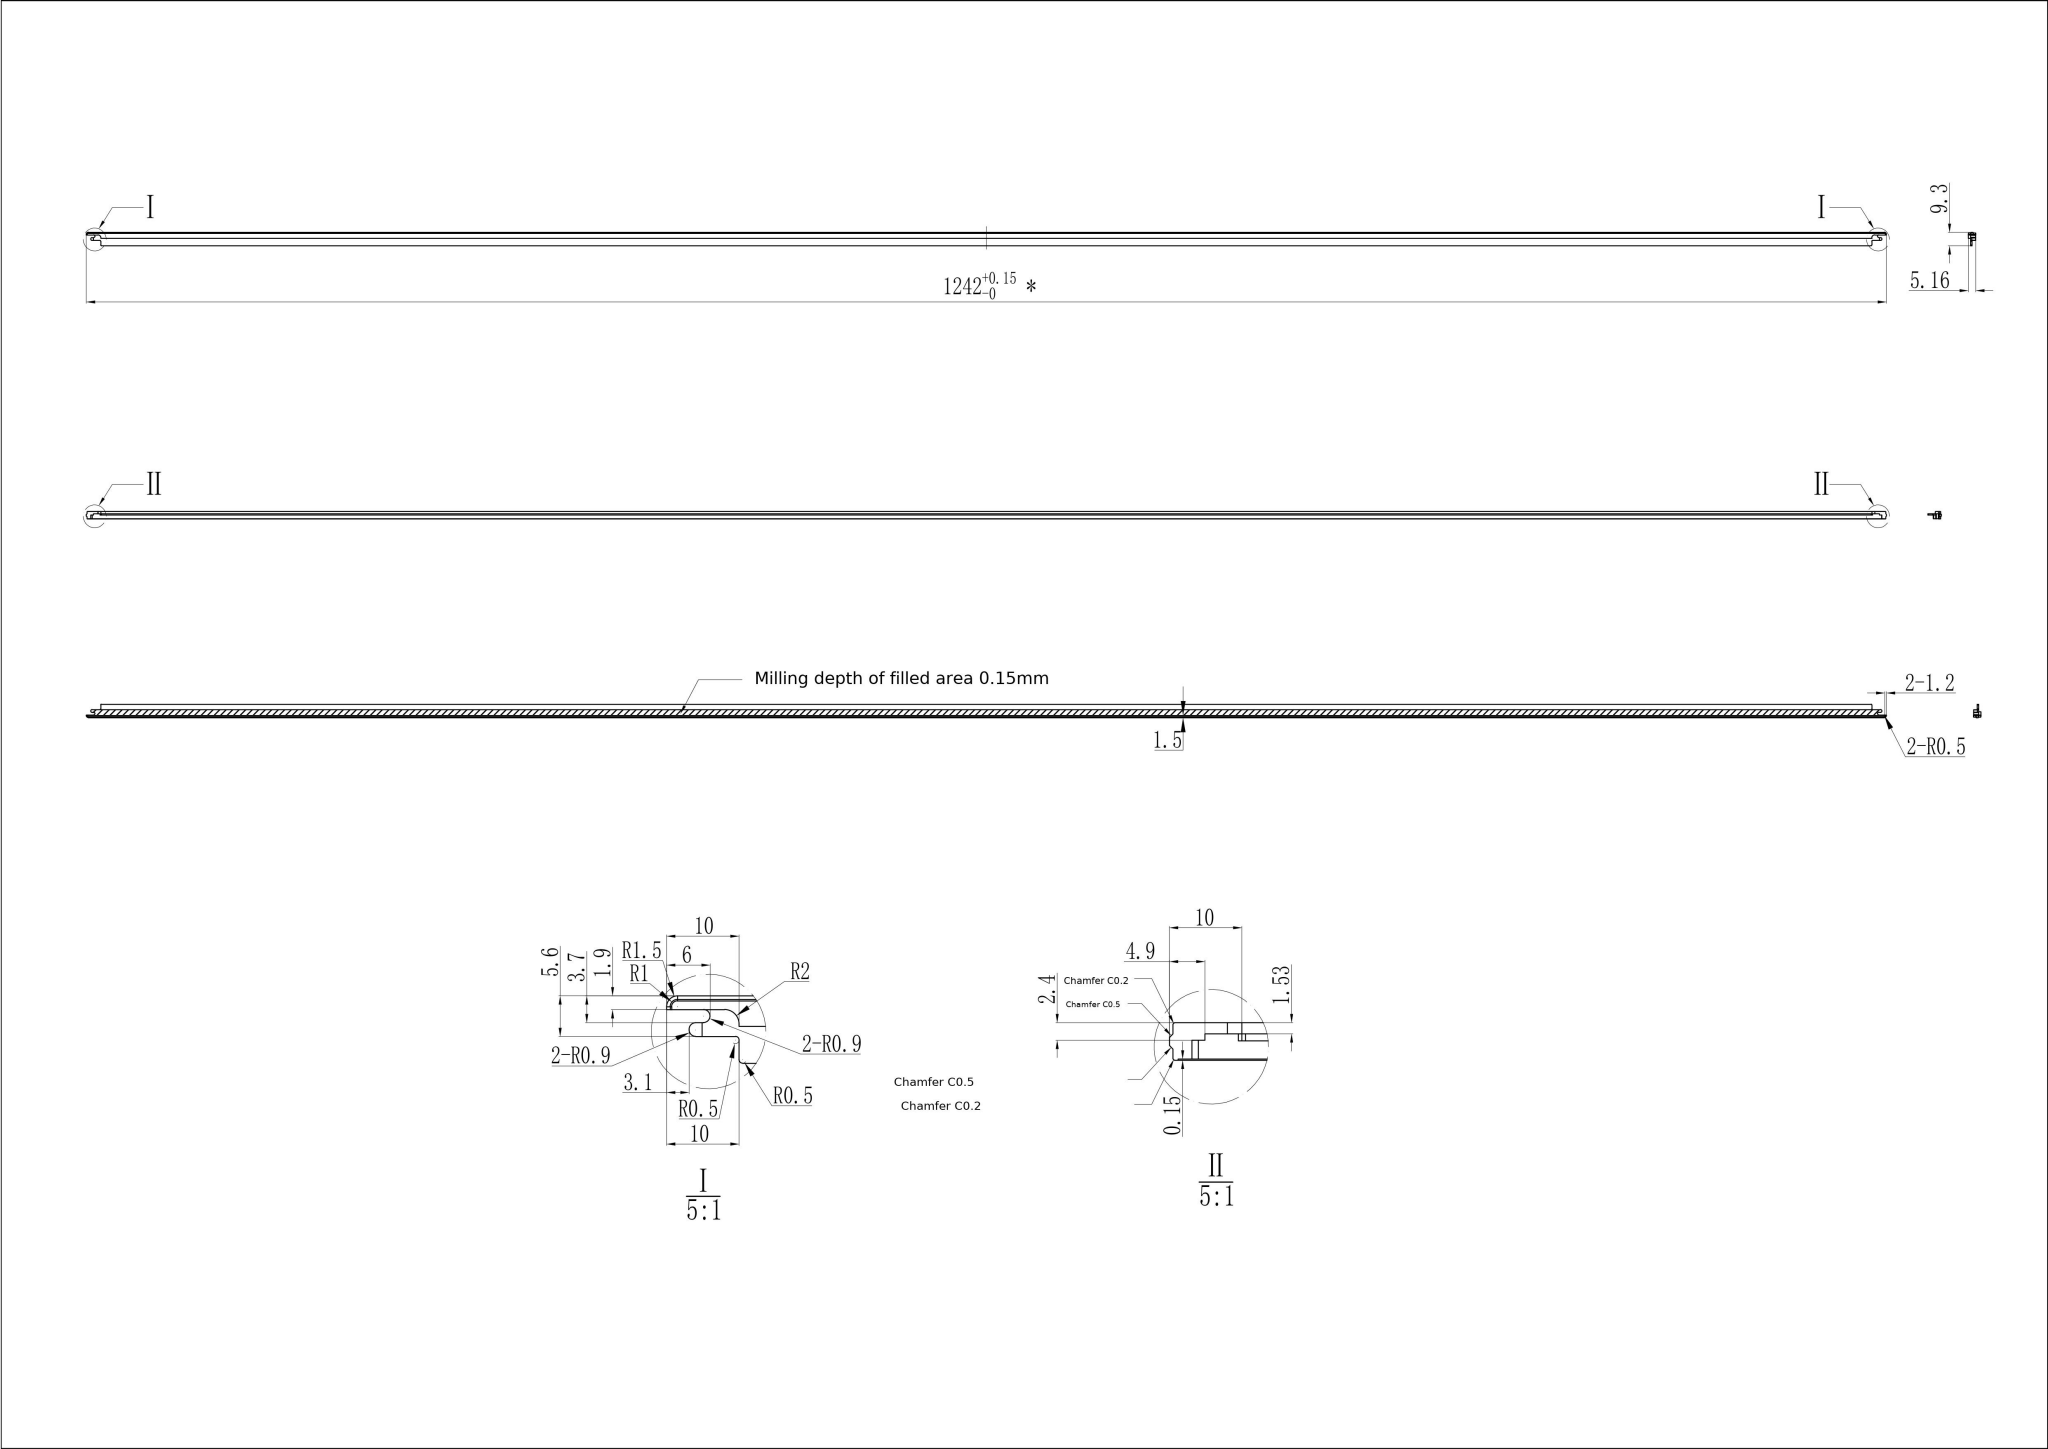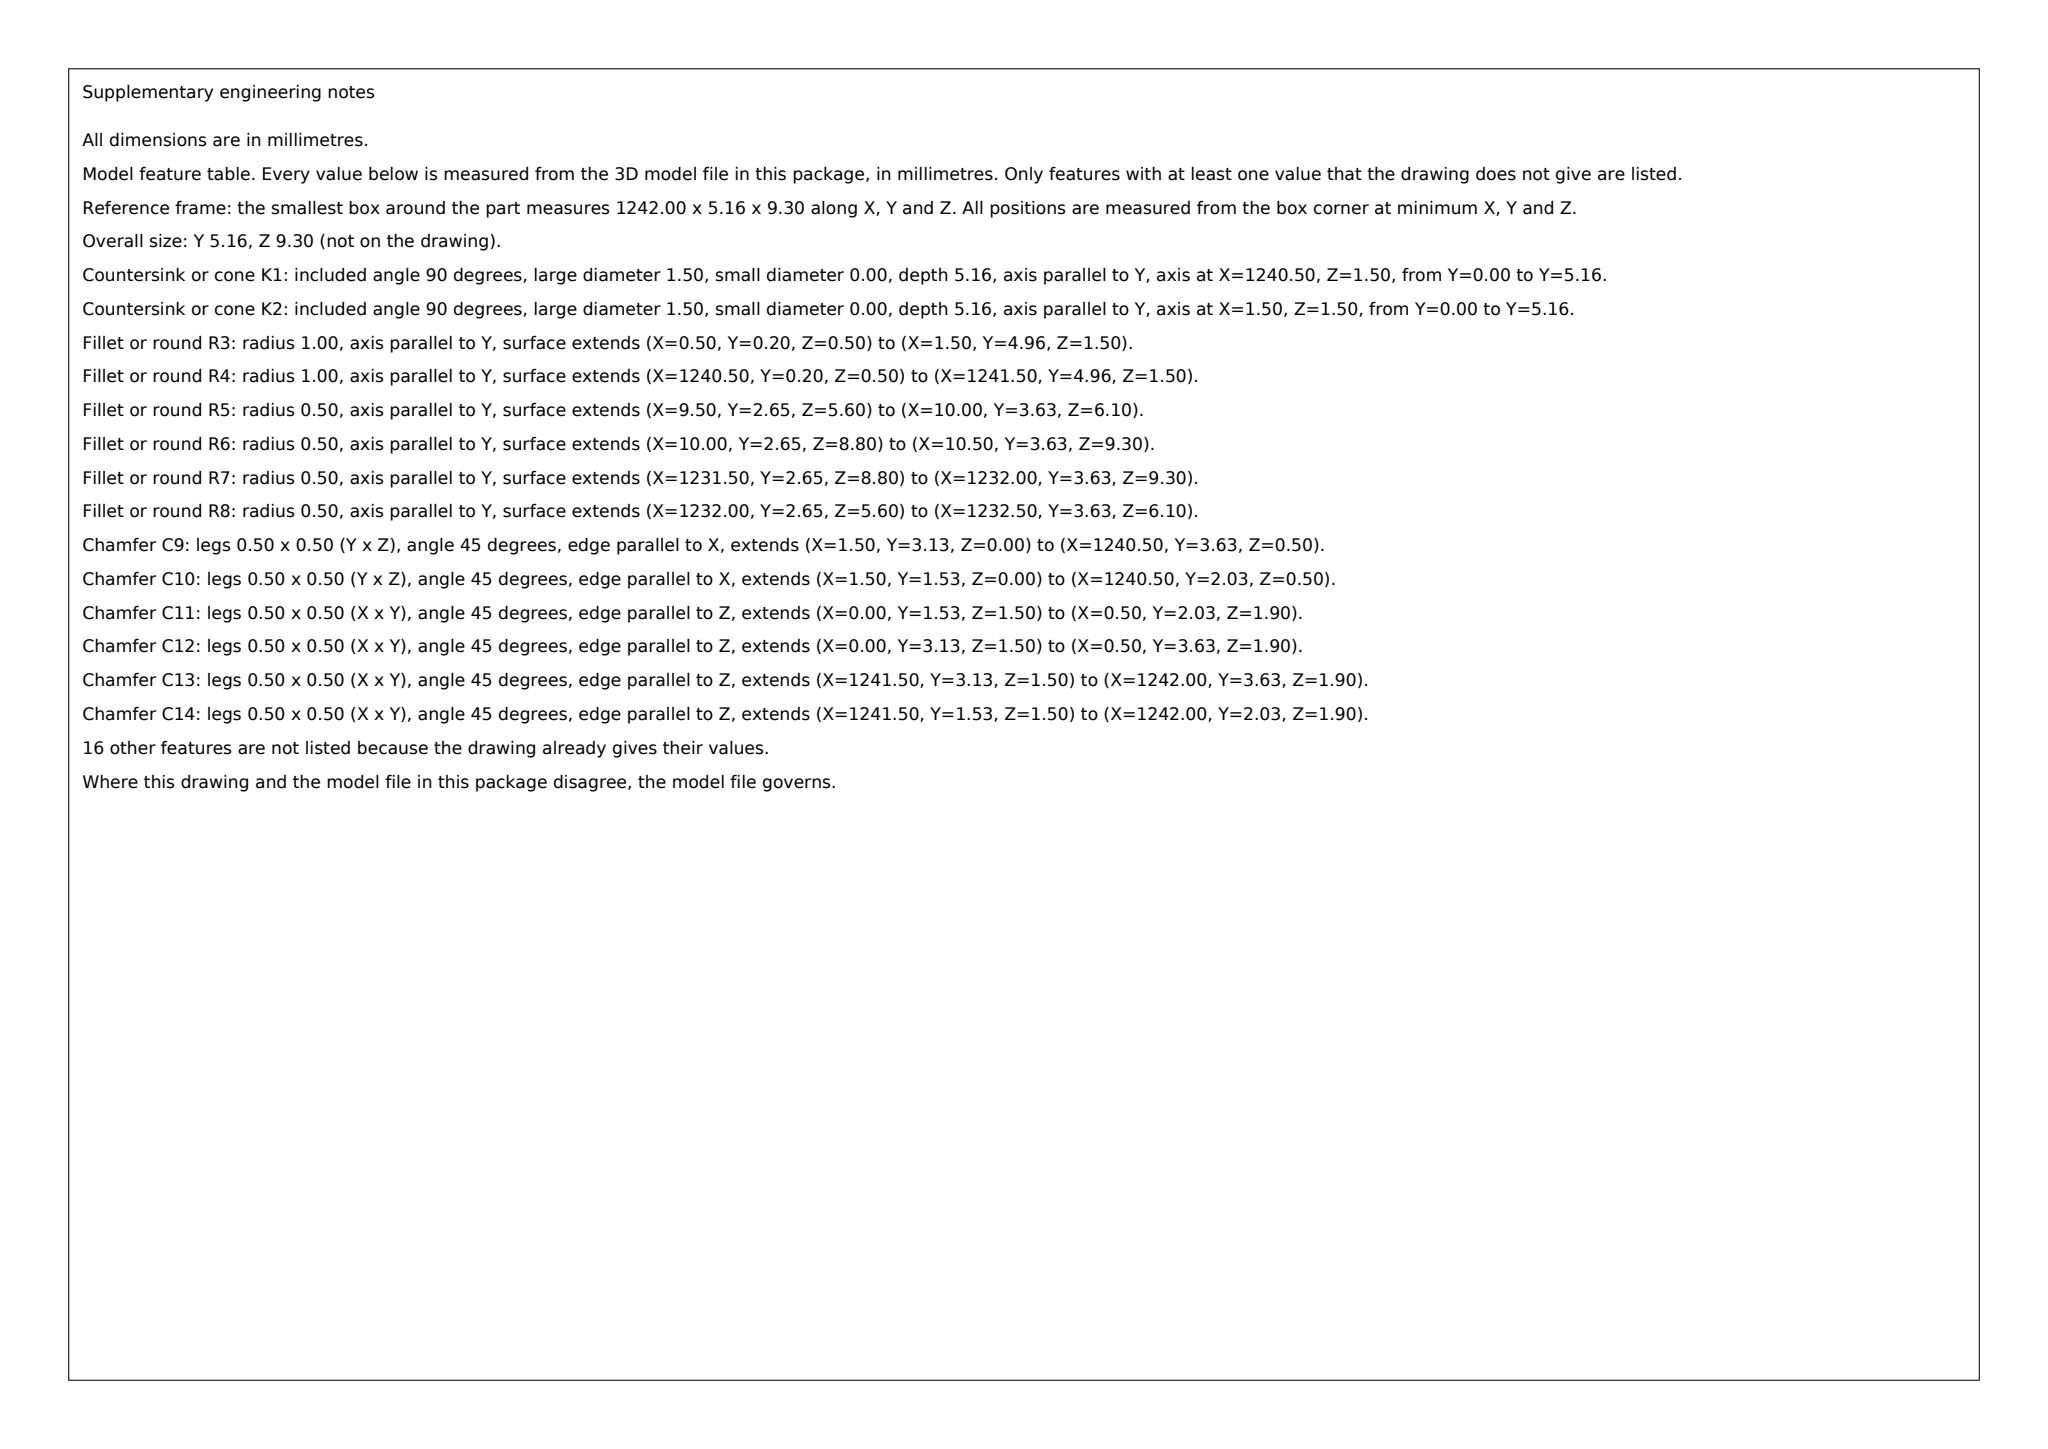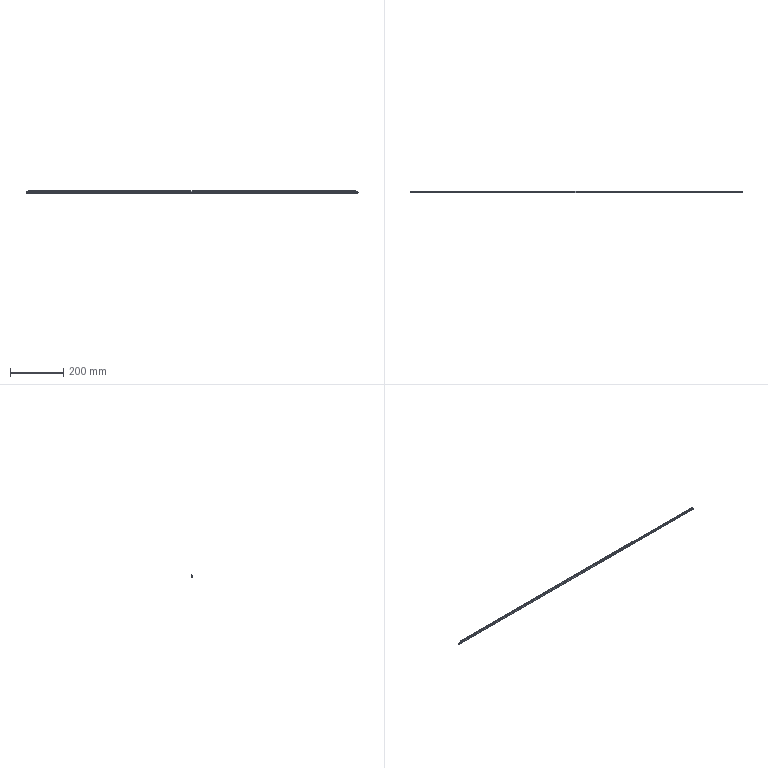Part | SolidWorks | mm | 1 solid | 74 faces | box 1242 x 5.16 x 9.3 mm | volume 34435 mm3 | plane 48 | cylinder 18 | cone 8 | commonest cylinder face diameters 0.4 x8 1 x4 2 x4 3 x2